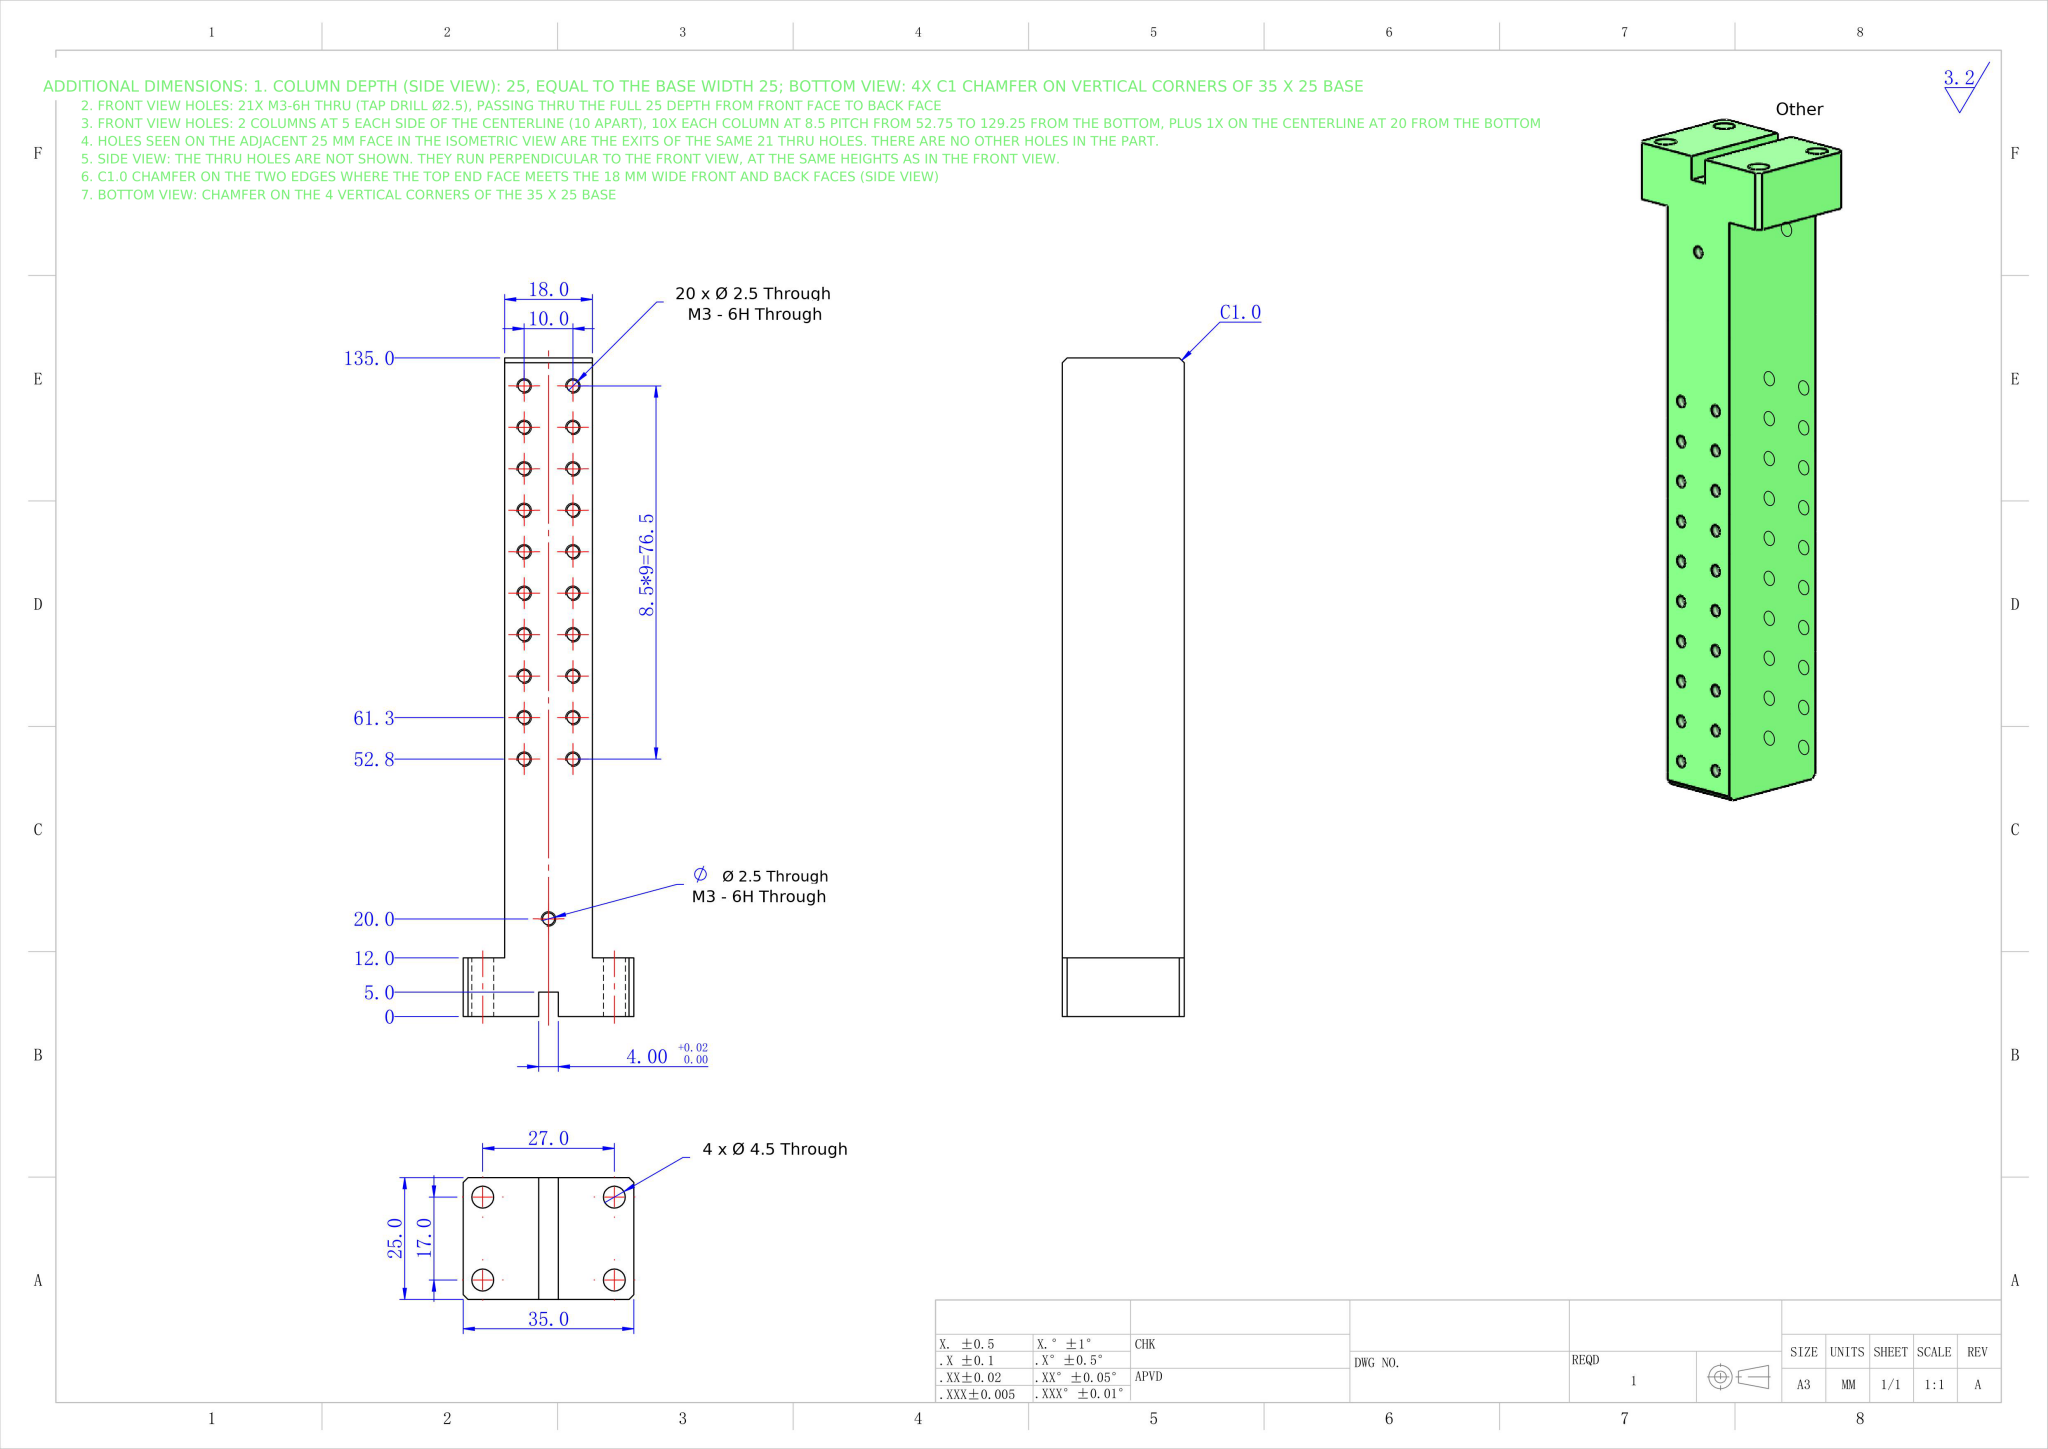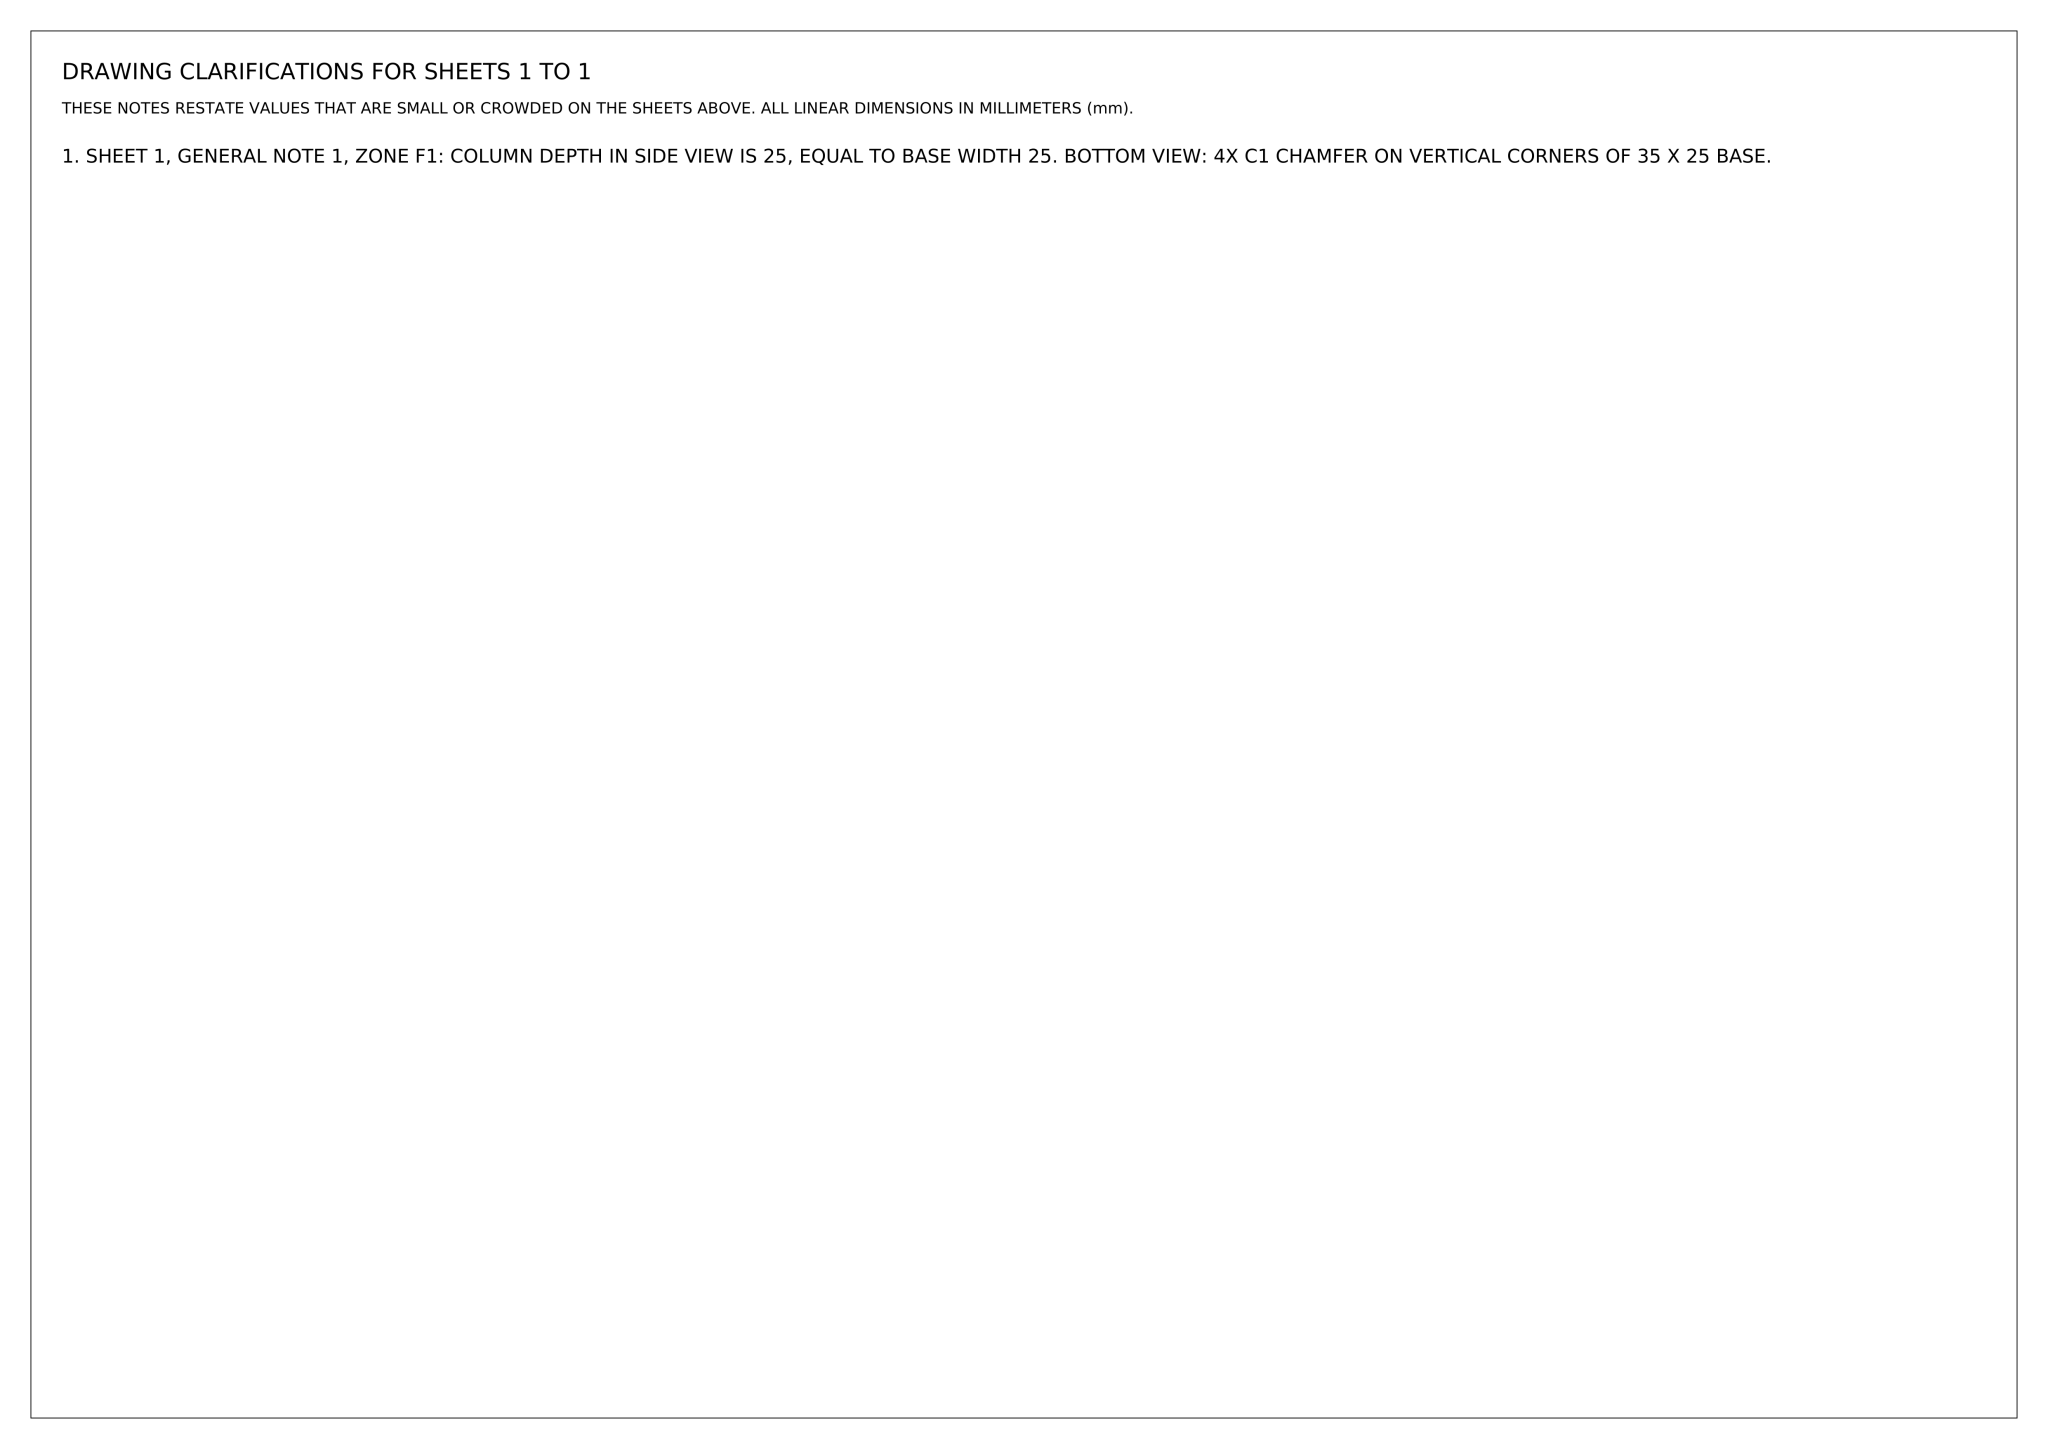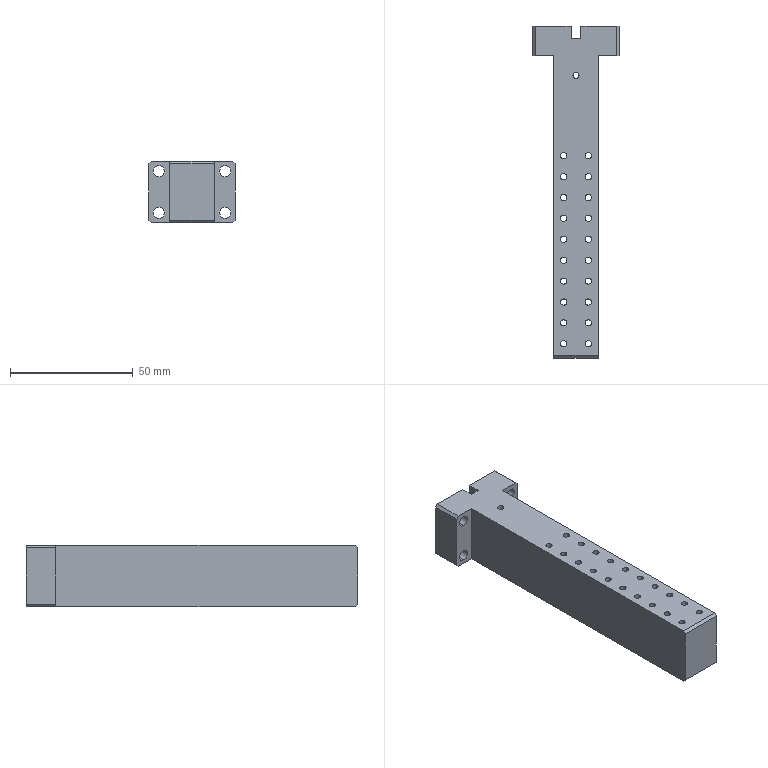Part | NX | mm | 1 solid | 70 faces | box 35 x 135 x 25 mm | volume 61968 mm3 | cylinder 50 | plane 20 | commonest cylinder face diameters 2.5 x42 4.5 x8